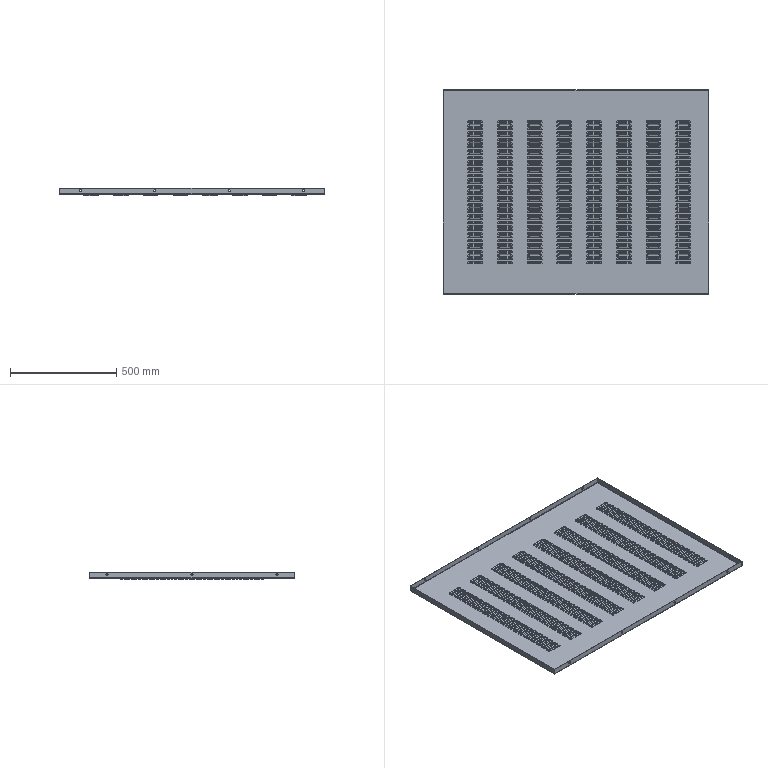Component | SolidWorks | 40RearCoverII-1 | 1 solid | 3266 faces | volume 2763290 mm3 | plane 1302 | torus 1280 | cylinder 676 | spline 8 | commonest cylinder face diameters 10 x348 14 x320 2 x4 6 x4